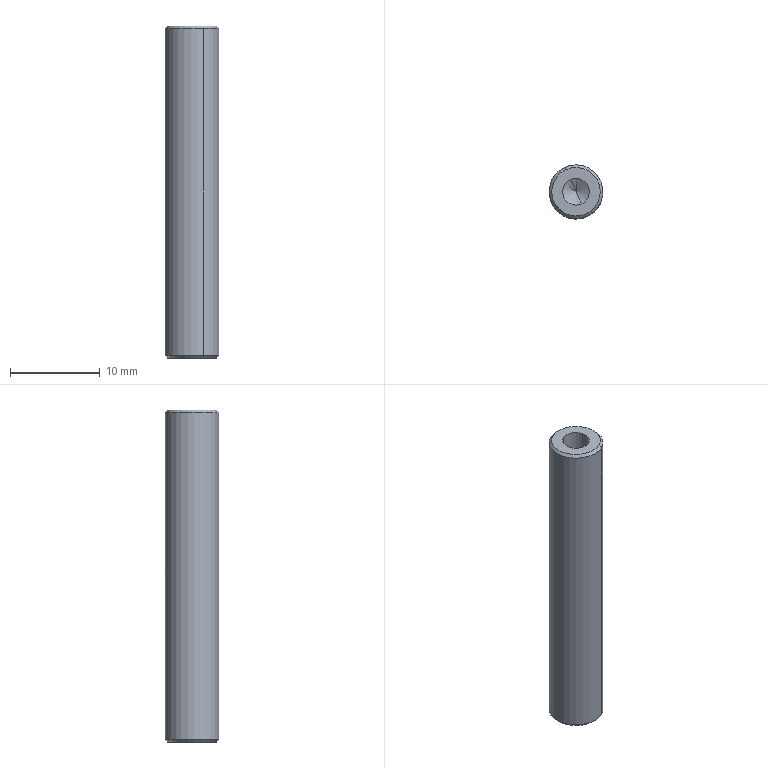Component | SolidWorks | WZH-20190520-F211StopBlockGuideRod-2 | 1 solid | 16 faces | box 6 x 6 x 37 mm | volume 906 mm3 | cone 8 | cylinder 6 | plane 2 | commonest cylinder face diameters 3 x4 6 x2 | material 45
build123d program:
from build123d import *

# Parameters (mm, degrees)
SKETCH1_R           = 3
BOSS_EXTRUDE1_DEPTH = 18.5
CHAMFER1_SIZE       = 0.3


with BuildPart() as part:
    # Sketch1 → Boss-Extrude1 (new, symmetric)
    with BuildSketch(Plane.XY):
        Circle(SKETCH1_R)
    extrude(amount=BOSS_EXTRUDE1_DEPTH, both=True)

    # Sketch3 → M3 Tapped Hole1 (revolve, cut)
    with BuildSketch(Plane(origin=(0, 0, 18.5), x_dir=(0, -1, 0), z_dir=(1, 0, 0))):
        Polygon((0, 0), (0, 10.401), (1.5, 9.5), (1.5, 0), align=None)
    m3_tapped_hole1 = revolve(axis=Axis((0, 0, 24.85), (0, 0, -1)), mode=Mode.SUBTRACT)

    # Mirror1: M3 Tapped Hole1 across plane
    add(m3_tapped_hole1.mirror(Plane.XY), mode=Mode.SUBTRACT)

    # Chamfer1
    chamfer1_edges = [part.edges().sort_by_distance(p)[0] for p in [
        (-3, 0, -18.5),
        (-3, 0, 18.5),
    ]]
    chamfer(chamfer1_edges, length=CHAMFER1_SIZE)


solid = part.part

# Placed as in the assembly
solid = solid.moved(Location((10, 5.5, -4.946), (0, 0, 0)))
STEP:
#1=COLOUR_RGB('',0.7922,0.8196,0.9333);
#2=FILL_AREA_STYLE_COLOUR('',#1);
#3=FILL_AREA_STYLE('',(#2));
#4=SURFACE_STYLE_FILL_AREA(#3);
#5=SURFACE_SIDE_STYLE('',(#4));
#6=SURFACE_STYLE_USAGE(.BOTH.,#5);
#7=PRESENTATION_STYLE_ASSIGNMENT((#6));
#8=CARTESIAN_POINT('',(0.3485,0.3128,0.5336));
#9=VERTEX_POINT('',#8);
#10=CARTESIAN_POINT('',(0.4389,0.1203,0.5336));
#11=VERTEX_POINT('',#10);
#12=CARTESIAN_POINT('',(0.3937,0.2165,0.5336));
#13=DIRECTION('',(0.,0.,1.));
#14=DIRECTION('',(-0.425,0.9052,0.));
#15=AXIS2_PLACEMENT_3D('',#12,#13,#14);
#16=CIRCLE('',#15,0.1063);
#17=EDGE_CURVE('',#9,#11,#16,.T.);
#18=ORIENTED_EDGE('',*,*,#17,.F.);
#19=CARTESIAN_POINT('',(0.3435,0.3234,0.5218));
#20=VERTEX_POINT('',#19);
#21=CARTESIAN_POINT('',(0.3485,0.3128,0.5336));
#22=DIRECTION('',(-0.3005,0.6401,-0.7071));
#23=VECTOR('',#22,39.37);
#24=LINE('',#21,#23);
#25=EDGE_CURVE('',#9,#20,#24,.T.);
#26=ORIENTED_EDGE('',*,*,#25,.T.);
#27=CARTESIAN_POINT('',(0.4439,0.1096,0.5218));
#28=VERTEX_POINT('',#27);
#29=CARTESIAN_POINT('',(0.3937,0.2165,0.5218));
#30=DIRECTION('',(0.,0.,-1.));
#31=DIRECTION('',(-0.425,0.9052,0.));
#32=AXIS2_PLACEMENT_3D('',#29,#30,#31);
#33=CIRCLE('',#32,0.1181);
#34=EDGE_CURVE('',#28,#20,#33,.T.);
#35=ORIENTED_EDGE('',*,*,#34,.F.);
#36=CARTESIAN_POINT('',(0.4389,0.1203,0.5336));
#37=DIRECTION('',(0.3005,-0.6401,-0.7071));
#38=VECTOR('',#37,39.37);
#39=LINE('',#36,#38);
#40=EDGE_CURVE('',#11,#28,#39,.T.);
#41=ORIENTED_EDGE('',*,*,#40,.F.);
#42=EDGE_LOOP('',(#18,#26,#35,#41));
#43=FACE_OUTER_BOUND('',#42,.T.);
#44=CARTESIAN_POINT('',(0.3937,0.2165,0.5336));
#45=DIRECTION('',(0.,0.,-1.));
#46=DIRECTION('',(0.425,-0.9052,0.));
#47=AXIS2_PLACEMENT_3D('',#44,#45,#46);
#48=CONICAL_SURFACE('',#47,0.1063,0.7854);
#49=ADVANCED_FACE('',(#43),#48,.T.);
#50=CARTESIAN_POINT('',(0.4389,0.1203,-0.9231));
#51=VERTEX_POINT('',#50);
#52=CARTESIAN_POINT('',(0.3485,0.3128,-0.9231));
#53=VERTEX_POINT('',#52);
#54=CARTESIAN_POINT('',(0.3937,0.2165,-0.9231));
#55=DIRECTION('',(0.,0.,-1.));
#56=DIRECTION('',(-0.425,0.9052,0.));
#57=AXIS2_PLACEMENT_3D('',#54,#55,#56);
#58=CIRCLE('',#57,0.1063);
#59=EDGE_CURVE('',#51,#53,#58,.T.);
#60=ORIENTED_EDGE('',*,*,#59,.F.);
#61=CARTESIAN_POINT('',(0.4439,0.1096,-0.9113));
#62=VERTEX_POINT('',#61);
#63=CARTESIAN_POINT('',(0.4439,0.1096,-0.9113));
#64=DIRECTION('',(0.3005,-0.6401,0.7071));
#65=VECTOR('',#64,39.37);
#66=LINE('',#63,#65);
#67=EDGE_CURVE('',#51,#62,#66,.T.);
#68=ORIENTED_EDGE('',*,*,#67,.T.);
#69=CARTESIAN_POINT('',(0.3435,0.3234,-0.9113));
#70=VERTEX_POINT('',#69);
#71=CARTESIAN_POINT('',(0.3937,0.2165,-0.9113));
#72=DIRECTION('',(0.,0.,1.));
#73=DIRECTION('',(-0.425,0.9052,0.));
#74=AXIS2_PLACEMENT_3D('',#71,#72,#73);
#75=CIRCLE('',#74,0.1181);
#76=EDGE_CURVE('',#70,#62,#75,.T.);
#77=ORIENTED_EDGE('',*,*,#76,.F.);
#78=CARTESIAN_POINT('',(0.3435,0.3234,-0.9113));
#79=DIRECTION('',(-0.3005,0.6401,0.7071));
#80=VECTOR('',#79,39.37);
#81=LINE('',#78,#80);
#82=EDGE_CURVE('',#53,#70,#81,.T.);
#83=ORIENTED_EDGE('',*,*,#82,.F.);
#84=EDGE_LOOP('',(#60,#68,#77,#83));
#85=FACE_OUTER_BOUND('',#84,.T.);
#86=CARTESIAN_POINT('',(0.3937,0.2165,-0.9113));
#87=DIRECTION('',(0.,0.,1.));
#88=DIRECTION('',(-0.425,0.9052,0.));
#89=AXIS2_PLACEMENT_3D('',#86,#87,#88);
#90=CONICAL_SURFACE('',#89,0.1181,0.7854);
#91=ADVANCED_FACE('',(#85),#90,.T.);
#92=CARTESIAN_POINT('',(0.3686,0.27,-0.5491));
#93=VERTEX_POINT('',#92);
#94=CARTESIAN_POINT('',(0.4188,0.1631,-0.5491));
#95=VERTEX_POINT('',#94);
#96=CARTESIAN_POINT('',(0.3937,0.2165,-0.5491));
#97=DIRECTION('',(0.,0.,-1.));
#98=DIRECTION('',(0.425,-0.9052,0.));
#99=AXIS2_PLACEMENT_3D('',#96,#97,#98);
#100=CIRCLE('',#99,0.05906);
#101=EDGE_CURVE('',#93,#95,#100,.T.);
#102=ORIENTED_EDGE('',*,*,#101,.F.);
#103=CARTESIAN_POINT('',(0.3686,0.27,-0.9231));
#104=VERTEX_POINT('',#103);
#105=CARTESIAN_POINT('',(0.3686,0.27,-0.9231));
#106=DIRECTION('',(0.,0.,-1.));
#107=VECTOR('',#106,39.37);
#108=LINE('',#105,#107);
#109=EDGE_CURVE('',#93,#104,#108,.T.);
#110=ORIENTED_EDGE('',*,*,#109,.T.);
#111=CARTESIAN_POINT('',(0.4188,0.1631,-0.9231));
#112=VERTEX_POINT('',#111);
#113=CARTESIAN_POINT('',(0.3937,0.2165,-0.9231));
#114=DIRECTION('',(0.,0.,-1.));
#115=DIRECTION('',(0.425,-0.9052,0.));
#116=AXIS2_PLACEMENT_3D('',#113,#114,#115);
#117=CIRCLE('',#116,0.05906);
#118=EDGE_CURVE('',#104,#112,#117,.T.);
#119=ORIENTED_EDGE('',*,*,#118,.T.);
#120=CARTESIAN_POINT('',(0.4188,0.1631,-0.9231));
#121=DIRECTION('',(0.,0.,-1.));
#122=VECTOR('',#121,39.37);
#123=LINE('',#120,#122);
#124=EDGE_CURVE('',#95,#112,#123,.T.);
#125=ORIENTED_EDGE('',*,*,#124,.F.);
#126=EDGE_LOOP('',(#102,#110,#119,#125));
#127=FACE_OUTER_BOUND('',#126,.T.);
#128=CARTESIAN_POINT('',(0.3937,0.2165,-0.9231));
#129=DIRECTION('',(0.,0.,-1.));
#130=DIRECTION('',(0.425,-0.9052,0.));
#131=AXIS2_PLACEMENT_3D('',#128,#129,#130);
#132=CYLINDRICAL_SURFACE('',#131,0.05906);
#133=ADVANCED_FACE('',(#127),#132,.F.);
#134=CARTESIAN_POINT('',(0.3937,0.2165,-0.5136));
#135=VERTEX_POINT('',#134);
#136=CARTESIAN_POINT('',(0.4188,0.1631,-0.5491));
#137=DIRECTION('',(0.3643,-0.7759,-0.515));
#138=VECTOR('',#137,39.37);
#139=LINE('',#136,#138);
#140=EDGE_CURVE('',#135,#95,#139,.T.);
#141=ORIENTED_EDGE('',*,*,#140,.F.);
#142=CARTESIAN_POINT('',(0.3686,0.27,-0.5491));
#143=DIRECTION('',(-0.3643,0.7759,-0.515));
#144=VECTOR('',#143,39.37);
#145=LINE('',#142,#144);
#146=EDGE_CURVE('',#135,#93,#145,.T.);
#147=ORIENTED_EDGE('',*,*,#146,.T.);
#148=ORIENTED_EDGE('',*,*,#101,.T.);
#149=EDGE_LOOP('',(#141,#147,#148));
#150=FACE_OUTER_BOUND('',#149,.T.);
#151=CARTESIAN_POINT('',(0.3937,0.2165,-0.5491));
#152=DIRECTION('',(0.,0.,-1.));
#153=DIRECTION('',(0.425,-0.9052,0.));
#154=AXIS2_PLACEMENT_3D('',#151,#152,#153);
#155=CONICAL_SURFACE('',#154,0.05906,1.03);
#156=ADVANCED_FACE('',(#150),#155,.F.);
#157=CARTESIAN_POINT('',(0.4188,0.1631,0.1596));
#158=VERTEX_POINT('',#157);
#159=CARTESIAN_POINT('',(0.3686,0.27,0.1596));
#160=VERTEX_POINT('',#159);
#161=CARTESIAN_POINT('',(0.3937,0.2165,0.1596));
#162=DIRECTION('',(0.,0.,1.));
#163=DIRECTION('',(-0.425,0.9052,0.));
#164=AXIS2_PLACEMENT_3D('',#161,#162,#163);
#165=CIRCLE('',#164,0.05906);
#166=EDGE_CURVE('',#158,#160,#165,.T.);
#167=ORIENTED_EDGE('',*,*,#166,.F.);
#168=CARTESIAN_POINT('',(0.4188,0.1631,0.5336));
#169=VERTEX_POINT('',#168);
#170=CARTESIAN_POINT('',(0.4188,0.1631,0.5336));
#171=DIRECTION('',(0.,0.,1.));
#172=VECTOR('',#171,39.37);
#173=LINE('',#170,#172);
#174=EDGE_CURVE('',#158,#169,#173,.T.);
#175=ORIENTED_EDGE('',*,*,#174,.T.);
#176=CARTESIAN_POINT('',(0.3686,0.27,0.5336));
#177=VERTEX_POINT('',#176);
#178=CARTESIAN_POINT('',(0.3937,0.2165,0.5336));
#179=DIRECTION('',(0.,0.,1.));
#180=DIRECTION('',(-0.425,0.9052,0.));
#181=AXIS2_PLACEMENT_3D('',#178,#179,#180);
#182=CIRCLE('',#181,0.05906);
#183=EDGE_CURVE('',#169,#177,#182,.T.);
#184=ORIENTED_EDGE('',*,*,#183,.T.);
#185=CARTESIAN_POINT('',(0.3686,0.27,0.5336));
#186=DIRECTION('',(0.,0.,1.));
#187=VECTOR('',#186,39.37);
#188=LINE('',#185,#187);
#189=EDGE_CURVE('',#160,#177,#188,.T.);
#190=ORIENTED_EDGE('',*,*,#189,.F.);
#191=EDGE_LOOP('',(#167,#175,#184,#190));
#192=FACE_OUTER_BOUND('',#191,.T.);
#193=CARTESIAN_POINT('',(0.3937,0.2165,0.5336));
#194=DIRECTION('',(0.,0.,1.));
#195=DIRECTION('',(-0.425,0.9052,0.));
#196=AXIS2_PLACEMENT_3D('',#193,#194,#195);
#197=CYLINDRICAL_SURFACE('',#196,0.05906);
#198=ADVANCED_FACE('',(#192),#197,.F.);
#199=CARTESIAN_POINT('',(0.3937,0.2165,0.1241));
#200=VERTEX_POINT('',#199);
#201=CARTESIAN_POINT('',(0.3686,0.27,0.1596));
#202=DIRECTION('',(-0.3643,0.7759,0.515));
#203=VECTOR('',#202,39.37);
#204=LINE('',#201,#203);
#205=EDGE_CURVE('',#200,#160,#204,.T.);
#206=ORIENTED_EDGE('',*,*,#205,.F.);
#207=CARTESIAN_POINT('',(0.4188,0.1631,0.1596));
#208=DIRECTION('',(0.3643,-0.7759,0.515));
#209=VECTOR('',#208,39.37);
#210=LINE('',#207,#209);
#211=EDGE_CURVE('',#200,#158,#210,.T.);
#212=ORIENTED_EDGE('',*,*,#211,.T.);
#213=ORIENTED_EDGE('',*,*,#166,.T.);
#214=EDGE_LOOP('',(#206,#212,#213));
#215=FACE_OUTER_BOUND('',#214,.T.);
#216=CARTESIAN_POINT('',(0.3937,0.2165,0.1596));
#217=DIRECTION('',(0.,0.,1.));
#218=DIRECTION('',(-0.425,0.9052,0.));
#219=AXIS2_PLACEMENT_3D('',#216,#217,#218);
#220=CONICAL_SURFACE('',#219,0.05906,1.03);
#221=ADVANCED_FACE('',(#215),#220,.F.);
#222=ORIENTED_EDGE('',*,*,#34,.T.);
#223=CARTESIAN_POINT('',(0.3435,0.3234,0.5336));
#224=DIRECTION('',(0.,0.,-1.));
#225=VECTOR('',#224,39.37);
#226=LINE('',#223,#225);
#227=EDGE_CURVE('',#20,#70,#226,.T.);
#228=ORIENTED_EDGE('',*,*,#227,.T.);
#229=ORIENTED_EDGE('',*,*,#76,.T.);
#230=CARTESIAN_POINT('',(0.4439,0.1096,0.5336));
#231=DIRECTION('',(0.,0.,-1.));
#232=VECTOR('',#231,39.37);
#233=LINE('',#230,#232);
#234=EDGE_CURVE('',#28,#62,#233,.T.);
#235=ORIENTED_EDGE('',*,*,#234,.F.);
#236=EDGE_LOOP('',(#222,#228,#229,#235));
#237=FACE_OUTER_BOUND('',#236,.T.);
#238=CARTESIAN_POINT('',(0.3937,0.2165,0.5336));
#239=DIRECTION('',(0.,0.,-1.));
#240=DIRECTION('',(0.425,-0.9052,0.));
#241=AXIS2_PLACEMENT_3D('',#238,#239,#240);
#242=CYLINDRICAL_SURFACE('',#241,0.1181);
#243=ADVANCED_FACE('',(#237),#242,.T.);
#244=ORIENTED_EDGE('',*,*,#227,.F.);
#245=CARTESIAN_POINT('',(0.3937,0.2165,0.5218));
#246=DIRECTION('',(0.,0.,-1.));
#247=DIRECTION('',(-0.425,0.9052,0.));
#248=AXIS2_PLACEMENT_3D('',#245,#246,#247);
#249=CIRCLE('',#248,0.1181);
#250=EDGE_CURVE('',#20,#28,#249,.T.);
#251=ORIENTED_EDGE('',*,*,#250,.T.);
#252=ORIENTED_EDGE('',*,*,#234,.T.);
#253=CARTESIAN_POINT('',(0.3937,0.2165,-0.9113));
#254=DIRECTION('',(0.,0.,1.));
#255=DIRECTION('',(-0.425,0.9052,0.));
#256=AXIS2_PLACEMENT_3D('',#253,#254,#255);
#257=CIRCLE('',#256,0.1181);
#258=EDGE_CURVE('',#62,#70,#257,.T.);
#259=ORIENTED_EDGE('',*,*,#258,.T.);
#260=EDGE_LOOP('',(#244,#251,#252,#259));
#261=FACE_OUTER_BOUND('',#260,.T.);
#262=CARTESIAN_POINT('',(0.3937,0.2165,0.5336));
#263=DIRECTION('',(0.,0.,-1.));
#264=DIRECTION('',(0.425,-0.9052,0.));
#265=AXIS2_PLACEMENT_3D('',#262,#263,#264);
#266=CYLINDRICAL_SURFACE('',#265,0.1181);
#267=ADVANCED_FACE('',(#261),#266,.T.);
#268=CARTESIAN_POINT('',(0.3937,0.2165,0.5336));
#269=DIRECTION('',(0.,0.,1.));
#270=DIRECTION('',(-0.425,0.9052,0.));
#271=AXIS2_PLACEMENT_3D('',#268,#269,#270);
#272=CIRCLE('',#271,0.1063);
#273=EDGE_CURVE('',#11,#9,#272,.T.);
#274=ORIENTED_EDGE('',*,*,#273,.T.);
#275=ORIENTED_EDGE('',*,*,#17,.T.);
#276=EDGE_LOOP('',(#274,#275));
#277=FACE_OUTER_BOUND('',#276,.T.);
#278=CARTESIAN_POINT('',(0.3937,0.2165,0.5336));
#279=DIRECTION('',(0.,0.,1.));
#280=DIRECTION('',(-0.425,0.9052,0.));
#281=AXIS2_PLACEMENT_3D('',#278,#279,#280);
#282=CIRCLE('',#281,0.05906);
#283=EDGE_CURVE('',#177,#169,#282,.T.);
#284=ORIENTED_EDGE('',*,*,#283,.F.);
#285=ORIENTED_EDGE('',*,*,#183,.F.);
#286=EDGE_LOOP('',(#284,#285));
#287=FACE_BOUND('',#286,.T.);
#288=CARTESIAN_POINT('',(0.3937,0.2165,0.5336));
#289=DIRECTION('',(0.,0.,1.));
#290=DIRECTION('',(-0.425,0.9052,0.));
#291=AXIS2_PLACEMENT_3D('',#288,#289,#290);
#292=PLANE('',#291);
#293=ADVANCED_FACE('',(#277,#287),#292,.T.);
#294=CARTESIAN_POINT('',(0.3937,0.2165,-0.9231));
#295=DIRECTION('',(0.,0.,-1.));
#296=DIRECTION('',(-0.425,0.9052,0.));
#297=AXIS2_PLACEMENT_3D('',#294,#295,#296);
#298=CIRCLE('',#297,0.1063);
#299=EDGE_CURVE('',#53,#51,#298,.T.);
#300=ORIENTED_EDGE('',*,*,#299,.T.);
#301=ORIENTED_EDGE('',*,*,#59,.T.);
#302=EDGE_LOOP('',(#300,#301));
#303=FACE_OUTER_BOUND('',#302,.T.);
#304=CARTESIAN_POINT('',(0.3937,0.2165,-0.9231));
#305=DIRECTION('',(0.,0.,-1.));
#306=DIRECTION('',(0.425,-0.9052,0.));
#307=AXIS2_PLACEMENT_3D('',#304,#305,#306);
#308=CIRCLE('',#307,0.05906);
#309=EDGE_CURVE('',#112,#104,#308,.T.);
#310=ORIENTED_EDGE('',*,*,#309,.F.);
#311=ORIENTED_EDGE('',*,*,#118,.F.);
#312=EDGE_LOOP('',(#310,#311));
#313=FACE_BOUND('',#312,.T.);
#314=CARTESIAN_POINT('',(0.3937,0.2165,-0.9231));
#315=DIRECTION('',(0.,0.,1.));
#316=DIRECTION('',(-0.425,0.9052,0.));
#317=AXIS2_PLACEMENT_3D('',#314,#315,#316);
#318=PLANE('',#317);
#319=ADVANCED_FACE('',(#303,#313),#318,.F.);
#320=ORIENTED_EDGE('',*,*,#211,.F.);
#321=ORIENTED_EDGE('',*,*,#205,.T.);
#322=CARTESIAN_POINT('',(0.3937,0.2165,0.1596));
#323=DIRECTION('',(0.,0.,1.));
#324=DIRECTION('',(-0.425,0.9052,0.));
#325=AXIS2_PLACEMENT_3D('',#322,#323,#324);
#326=CIRCLE('',#325,0.05906);
#327=EDGE_CURVE('',#160,#158,#326,.T.);
#328=ORIENTED_EDGE('',*,*,#327,.T.);
#329=EDGE_LOOP('',(#320,#321,#328));
#330=FACE_OUTER_BOUND('',#329,.T.);
#331=CARTESIAN_POINT('',(0.3937,0.2165,0.1596));
#332=DIRECTION('',(0.,0.,1.));
#333=DIRECTION('',(-0.425,0.9052,0.));
#334=AXIS2_PLACEMENT_3D('',#331,#332,#333);
#335=CONICAL_SURFACE('',#334,0.05906,1.03);
#336=ADVANCED_FACE('',(#330),#335,.F.);
#337=ORIENTED_EDGE('',*,*,#174,.F.);
#338=ORIENTED_EDGE('',*,*,#327,.F.);
#339=ORIENTED_EDGE('',*,*,#189,.T.);
#340=ORIENTED_EDGE('',*,*,#283,.T.);
#341=EDGE_LOOP('',(#337,#338,#339,#340));
#342=FACE_OUTER_BOUND('',#341,.T.);
#343=CARTESIAN_POINT('',(0.3937,0.2165,0.5336));
#344=DIRECTION('',(0.,0.,1.));
#345=DIRECTION('',(-0.425,0.9052,0.));
#346=AXIS2_PLACEMENT_3D('',#343,#344,#345);
#347=CYLINDRICAL_SURFACE('',#346,0.05906);
#348=ADVANCED_FACE('',(#342),#347,.F.);
#349=ORIENTED_EDGE('',*,*,#146,.F.);
#350=ORIENTED_EDGE('',*,*,#140,.T.);
#351=CARTESIAN_POINT('',(0.3937,0.2165,-0.5491));
#352=DIRECTION('',(0.,0.,-1.));
#353=DIRECTION('',(0.425,-0.9052,0.));
#354=AXIS2_PLACEMENT_3D('',#351,#352,#353);
#355=CIRCLE('',#354,0.05906);
#356=EDGE_CURVE('',#95,#93,#355,.T.);
#357=ORIENTED_EDGE('',*,*,#356,.T.);
#358=EDGE_LOOP('',(#349,#350,#357));
#359=FACE_OUTER_BOUND('',#358,.T.);
#360=CARTESIAN_POINT('',(0.3937,0.2165,-0.5491));
#361=DIRECTION('',(0.,0.,-1.));
#362=DIRECTION('',(0.425,-0.9052,0.));
#363=AXIS2_PLACEMENT_3D('',#360,#361,#362);
#364=CONICAL_SURFACE('',#363,0.05906,1.03);
#365=ADVANCED_FACE('',(#359),#364,.F.);
#366=ORIENTED_EDGE('',*,*,#109,.F.);
#367=ORIENTED_EDGE('',*,*,#356,.F.);
#368=ORIENTED_EDGE('',*,*,#124,.T.);
#369=ORIENTED_EDGE('',*,*,#309,.T.);
#370=EDGE_LOOP('',(#366,#367,#368,#369));
#371=FACE_OUTER_BOUND('',#370,.T.);
#372=CARTESIAN_POINT('',(0.3937,0.2165,-0.9231));
#373=DIRECTION('',(0.,0.,-1.));
#374=DIRECTION('',(0.425,-0.9052,0.));
#375=AXIS2_PLACEMENT_3D('',#372,#373,#374);
#376=CYLINDRICAL_SURFACE('',#375,0.05906);
#377=ADVANCED_FACE('',(#371),#376,.F.);
#378=ORIENTED_EDGE('',*,*,#67,.F.);
#379=ORIENTED_EDGE('',*,*,#299,.F.);
#380=ORIENTED_EDGE('',*,*,#82,.T.);
#381=ORIENTED_EDGE('',*,*,#258,.F.);
#382=EDGE_LOOP('',(#378,#379,#380,#381));
#383=FACE_OUTER_BOUND('',#382,.T.);
#384=CARTESIAN_POINT('',(0.3937,0.2165,-0.9113));
#385=DIRECTION('',(0.,0.,1.));
#386=DIRECTION('',(-0.425,0.9052,0.));
#387=AXIS2_PLACEMENT_3D('',#384,#385,#386);
#388=CONICAL_SURFACE('',#387,0.1181,0.7854);
#389=ADVANCED_FACE('',(#383),#388,.T.);
#390=ORIENTED_EDGE('',*,*,#25,.F.);
#391=ORIENTED_EDGE('',*,*,#273,.F.);
#392=ORIENTED_EDGE('',*,*,#40,.T.);
#393=ORIENTED_EDGE('',*,*,#250,.F.);
#394=EDGE_LOOP('',(#390,#391,#392,#393));
#395=FACE_OUTER_BOUND('',#394,.T.);
#396=CARTESIAN_POINT('',(0.3937,0.2165,0.5336));
#397=DIRECTION('',(0.,0.,-1.));
#398=DIRECTION('',(0.425,-0.9052,0.));
#399=AXIS2_PLACEMENT_3D('',#396,#397,#398);
#400=CONICAL_SURFACE('',#399,0.1063,0.7854);
#401=ADVANCED_FACE('',(#395),#400,.T.);
#402=CLOSED_SHELL('',(#49,#91,#133,#156,#198,#221,#243,#267,#293,#319,#336,#348,#365,#377,#389,#401));
#403=MANIFOLD_SOLID_BREP('',#402);
#404=STYLED_ITEM('',(#7),#403);
#405=(LENGTH_UNIT()NAMED_UNIT(*)SI_UNIT($,.METRE.));
#406=LENGTH_MEASURE_WITH_UNIT(LENGTH_MEASURE(0.0254),#405);
#407=DIMENSIONAL_EXPONENTS(1.,0.,0.,0.,0.,0.,0.);
#408=(CONVERSION_BASED_UNIT('',#406)LENGTH_UNIT()NAMED_UNIT(#407));
#409=UNCERTAINTY_MEASURE_WITH_UNIT(LENGTH_MEASURE(0.00001),#408,'','');
#410=(NAMED_UNIT(*)PLANE_ANGLE_UNIT()SI_UNIT($,.RADIAN.));
#411=(NAMED_UNIT(*)SI_UNIT($,.STERADIAN.)SOLID_ANGLE_UNIT());
#412=(GEOMETRIC_REPRESENTATION_CONTEXT(3)GLOBAL_UNCERTAINTY_ASSIGNED_CONTEXT((#409))GLOBAL_UNIT_ASSIGNED_CONTEXT((#408,#410,#411))REPRESENTATION_CONTEXT('',''));
#413=MECHANICAL_DESIGN_GEOMETRIC_PRESENTATION_REPRESENTATION('',(#404),#412);
#414=CARTESIAN_POINT('',(0.,0.,0.));
#415=DIRECTION('',(0.,0.,1.));
#416=DIRECTION('',(1.,0.,0.));
#417=AXIS2_PLACEMENT_3D('',#414,#415,#416);
#418=(LENGTH_UNIT()NAMED_UNIT(*)SI_UNIT($,.METRE.));
#419=LENGTH_MEASURE_WITH_UNIT(LENGTH_MEASURE(0.0254),#418);
#420=DIMENSIONAL_EXPONENTS(1.,0.,0.,0.,0.,0.,0.);
#421=(CONVERSION_BASED_UNIT('',#419)LENGTH_UNIT()NAMED_UNIT(#420));
#422=UNCERTAINTY_MEASURE_WITH_UNIT(LENGTH_MEASURE(0.00001),#421,'','');
#423=(NAMED_UNIT(*)PLANE_ANGLE_UNIT()SI_UNIT($,.RADIAN.));
#424=(NAMED_UNIT(*)SI_UNIT($,.STERADIAN.)SOLID_ANGLE_UNIT());
#425=(GEOMETRIC_REPRESENTATION_CONTEXT(3)GLOBAL_UNCERTAINTY_ASSIGNED_CONTEXT((#422))GLOBAL_UNIT_ASSIGNED_CONTEXT((#421,#423,#424))REPRESENTATION_CONTEXT('',''));
#426=ADVANCED_BREP_SHAPE_REPRESENTATION('',(#403,#417),#425);
#427=PRESENTATION_LAYER_ASSIGNMENT('','',(#404));